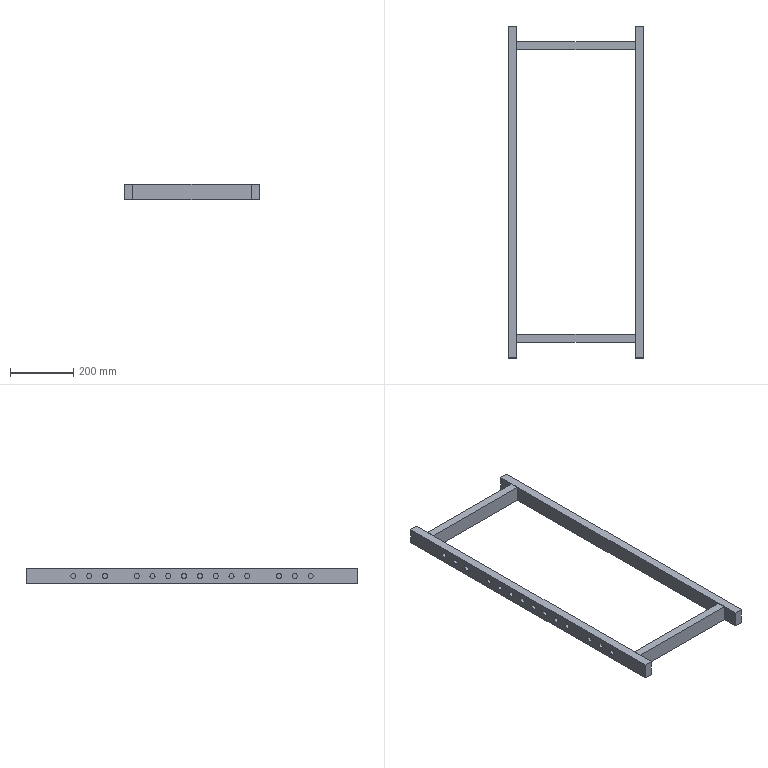Component | SolidWorks | Part12-1 | 4 solids | 52 faces | volume 3698999 mm3 | cylinder 28 | plane 24 | commonest cylinder face diameters 16 x28